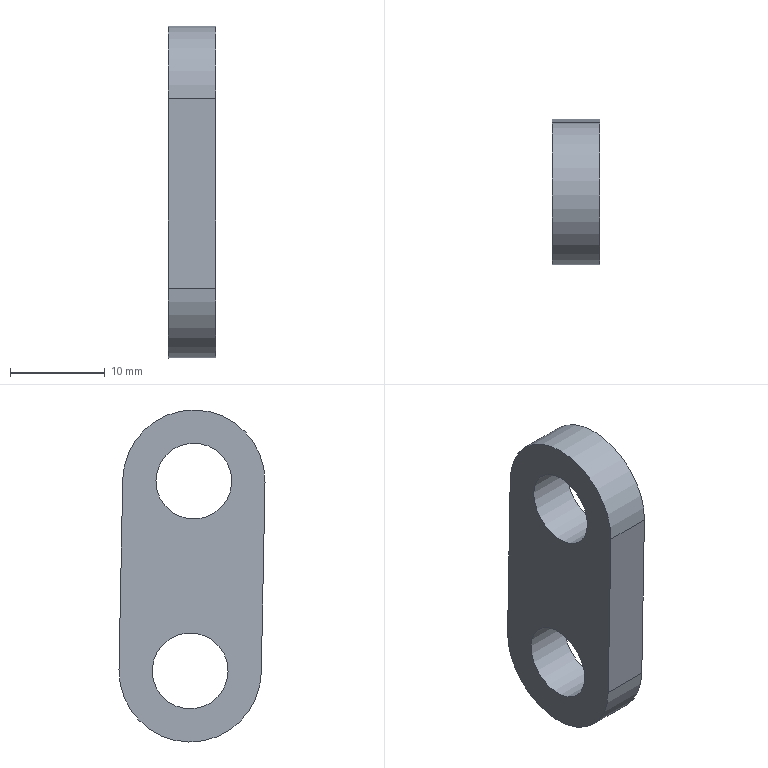Component | NX | LINK1_2 | 1 solid | 8 faces | box 5 x 15.39 x 35 mm | volume 1881 mm3 | plane 4 | cylinder 4 | commonest cylinder face diameters 15 x2 8 x2
STEP:
#1=CARTESIAN_POINT('',(0.,0.,0.));
#2=DIRECTION('',(0.,0.,1.));
#3=DIRECTION('',(1.,0.,0.));
#4=AXIS2_PLACEMENT_3D('',#1,#2,#3);
#5=CARTESIAN_POINT('',(4.61,-32.598,-197.455));
#6=VERTEX_POINT('',#5);
#7=CARTESIAN_POINT('',(4.61,-28.599,-197.377));
#8=DIRECTION('',(-1.,0.,0.));
#9=DIRECTION('',(0.,-0.9998,-0.01963));
#10=AXIS2_PLACEMENT_3D('',#7,#8,#9);
#11=CIRCLE('',#10,4.);
#12=CARTESIAN_POINT('',(4.61,-28.403,-207.375));
#13=DIRECTION('',(1.,0.,0.));
#14=DIRECTION('',(0.,0.9998,0.01963));
#15=AXIS2_PLACEMENT_3D('',#12,#13,#14);
#16=PLANE('',#15);
#17=CARTESIAN_POINT('',(-4.,10.));
#18=CARTESIAN_POINT('',(-4.,16.928));
#19=CARTESIAN_POINT('',(2.,13.464));
#20=CARTESIAN_POINT('',(8.,10.));
#21=CARTESIAN_POINT('',(2.,6.536));
#22=CARTESIAN_POINT('',(-4.,3.072));
#23=CARTESIAN_POINT('',(-4.,10.));
#24=(BOUNDED_CURVE()B_SPLINE_CURVE(2,(#17,#18,#19,#20,#21,#22,#23),.UNSPECIFIED.,.T.,.F.)B_SPLINE_CURVE_WITH_KNOTS((1,2,2,2,2,1),(-2.094,0.,2.094,4.189,6.283,8.378),.UNSPECIFIED.)CURVE()GEOMETRIC_REPRESENTATION_ITEM()RATIONAL_B_SPLINE_CURVE((1.,0.5,1.,0.5,1.,0.5,1.))REPRESENTATION_ITEM(''));
#25=(GEOMETRIC_REPRESENTATION_CONTEXT(2)PARAMETRIC_REPRESENTATION_CONTEXT()REPRESENTATION_CONTEXT('',''));
#26=DEFINITIONAL_REPRESENTATION('',(#24),#25);
#27=PCURVE('',#16,#26);
#28=CARTESIAN_POINT('',(4.61,-28.599,-197.377));
#29=DIRECTION('',(-1.,0.,0.));
#30=DIRECTION('',(0.,-0.9998,-0.01963));
#31=AXIS2_PLACEMENT_3D('',#28,#29,#30);
#32=CYLINDRICAL_SURFACE('',#31,4.);
#33=CARTESIAN_POINT('',(0.,0.));
#34=DIRECTION('',(1.,0.));
#35=VECTOR('',#34,1.);
#36=LINE('',#33,#35);
#37=(GEOMETRIC_REPRESENTATION_CONTEXT(2)PARAMETRIC_REPRESENTATION_CONTEXT()REPRESENTATION_CONTEXT('',''));
#38=DEFINITIONAL_REPRESENTATION('',(#36),#37);
#39=PCURVE('',#32,#38);
#40=SURFACE_CURVE('',#11,(#27,#39),.PCURVE_S1.);
#41=EDGE_CURVE('',#6,#6,#40,.T.);
#42=ORIENTED_EDGE('',*,*,#41,.T.);
#43=EDGE_LOOP('',(#42));
#44=FACE_BOUND('',#43,.T.);
#45=CARTESIAN_POINT('',(4.61,-32.206,-217.451));
#46=VERTEX_POINT('',#45);
#47=CARTESIAN_POINT('',(4.61,-28.206,-217.373));
#48=DIRECTION('',(-1.,0.,0.));
#49=DIRECTION('',(0.,-0.9998,-0.01963));
#50=AXIS2_PLACEMENT_3D('',#47,#48,#49);
#51=CIRCLE('',#50,4.);
#52=CARTESIAN_POINT('',(-4.,-10.));
#53=CARTESIAN_POINT('',(-4.,-3.072));
#54=CARTESIAN_POINT('',(2.,-6.536));
#55=CARTESIAN_POINT('',(8.,-10.));
#56=CARTESIAN_POINT('',(2.,-13.464));
#57=CARTESIAN_POINT('',(-4.,-16.928));
#58=CARTESIAN_POINT('',(-4.,-10.));
#59=(BOUNDED_CURVE()B_SPLINE_CURVE(2,(#52,#53,#54,#55,#56,#57,#58),.UNSPECIFIED.,.T.,.F.)B_SPLINE_CURVE_WITH_KNOTS((1,2,2,2,2,1),(-2.094,0.,2.094,4.189,6.283,8.378),.UNSPECIFIED.)CURVE()GEOMETRIC_REPRESENTATION_ITEM()RATIONAL_B_SPLINE_CURVE((1.,0.5,1.,0.5,1.,0.5,1.))REPRESENTATION_ITEM(''));
#60=(GEOMETRIC_REPRESENTATION_CONTEXT(2)PARAMETRIC_REPRESENTATION_CONTEXT()REPRESENTATION_CONTEXT('',''));
#61=DEFINITIONAL_REPRESENTATION('',(#59),#60);
#62=PCURVE('',#16,#61);
#63=CARTESIAN_POINT('',(4.61,-28.206,-217.373));
#64=DIRECTION('',(-1.,0.,0.));
#65=DIRECTION('',(0.,-0.9998,-0.01963));
#66=AXIS2_PLACEMENT_3D('',#63,#64,#65);
#67=CYLINDRICAL_SURFACE('',#66,4.);
#68=CARTESIAN_POINT('',(0.,0.));
#69=DIRECTION('',(1.,0.));
#70=VECTOR('',#69,1.);
#71=LINE('',#68,#70);
#72=(GEOMETRIC_REPRESENTATION_CONTEXT(2)PARAMETRIC_REPRESENTATION_CONTEXT()REPRESENTATION_CONTEXT('',''));
#73=DEFINITIONAL_REPRESENTATION('',(#71),#72);
#74=PCURVE('',#67,#73);
#75=SURFACE_CURVE('',#51,(#62,#74),.PCURVE_S1.);
#76=EDGE_CURVE('',#46,#46,#75,.T.);
#77=ORIENTED_EDGE('',*,*,#76,.T.);
#78=EDGE_LOOP('',(#77));
#79=FACE_BOUND('',#78,.T.);
#80=CARTESIAN_POINT('',(4.61,-21.1,-197.229));
#81=VERTEX_POINT('',#80);
#82=CARTESIAN_POINT('',(4.61,-36.098,-197.524));
#83=VERTEX_POINT('',#82);
#84=CARTESIAN_POINT('',(4.61,-28.599,-197.377));
#85=DIRECTION('',(1.,0.,0.));
#86=DIRECTION('',(0.,0.9998,0.01963));
#87=AXIS2_PLACEMENT_3D('',#84,#85,#86);
#88=CIRCLE('',#87,7.5);
#89=CARTESIAN_POINT('',(0.,10.));
#90=DIRECTION('',(1.,0.));
#91=AXIS2_PLACEMENT_2D('',#89,#90);
#92=CIRCLE('',#91,7.5);
#93=(GEOMETRIC_REPRESENTATION_CONTEXT(2)PARAMETRIC_REPRESENTATION_CONTEXT()REPRESENTATION_CONTEXT('',''));
#94=DEFINITIONAL_REPRESENTATION('',(#92),#93);
#95=PCURVE('',#16,#94);
#96=CARTESIAN_POINT('',(-0.3896,-28.599,-197.377));
#97=DIRECTION('',(1.,0.,0.));
#98=DIRECTION('',(0.,0.9998,0.01963));
#99=AXIS2_PLACEMENT_3D('',#96,#97,#98);
#100=CYLINDRICAL_SURFACE('',#99,7.5);
#101=CARTESIAN_POINT('',(0.,5.));
#102=DIRECTION('',(1.,0.));
#103=VECTOR('',#102,1.);
#104=LINE('',#101,#103);
#105=(GEOMETRIC_REPRESENTATION_CONTEXT(2)PARAMETRIC_REPRESENTATION_CONTEXT()REPRESENTATION_CONTEXT('',''));
#106=DEFINITIONAL_REPRESENTATION('',(#104),#105);
#107=PCURVE('',#100,#106);
#108=SURFACE_CURVE('',#88,(#95,#107),.PCURVE_S1.);
#109=EDGE_CURVE('',#81,#83,#108,.T.);
#110=ORIENTED_EDGE('',*,*,#109,.T.);
#111=CARTESIAN_POINT('',(4.61,-35.705,-217.52));
#112=VERTEX_POINT('',#111);
#113=CARTESIAN_POINT('',(4.61,-35.901,-207.522));
#114=DIRECTION('',(0.,-0.01963,0.9998));
#115=VECTOR('',#114,1.);
#116=LINE('',#113,#115);
#117=CARTESIAN_POINT('',(-7.5,-0.));
#118=DIRECTION('',(0.,1.));
#119=VECTOR('',#118,1.);
#120=LINE('',#117,#119);
#121=(GEOMETRIC_REPRESENTATION_CONTEXT(2)PARAMETRIC_REPRESENTATION_CONTEXT()REPRESENTATION_CONTEXT('',''));
#122=DEFINITIONAL_REPRESENTATION('',(#120),#121);
#123=PCURVE('',#16,#122);
#124=CARTESIAN_POINT('',(-0.3896,-35.901,-207.522));
#125=DIRECTION('',(0.,-0.9998,-0.01963));
#126=DIRECTION('',(1.,0.,0.));
#127=AXIS2_PLACEMENT_3D('',#124,#125,#126);
#128=PLANE('',#127);
#129=CARTESIAN_POINT('',(5.,0.));
#130=DIRECTION('',(0.,1.));
#131=VECTOR('',#130,1.);
#132=LINE('',#129,#131);
#133=(GEOMETRIC_REPRESENTATION_CONTEXT(2)PARAMETRIC_REPRESENTATION_CONTEXT()REPRESENTATION_CONTEXT('',''));
#134=DEFINITIONAL_REPRESENTATION('',(#132),#133);
#135=PCURVE('',#128,#134);
#136=SURFACE_CURVE('',#116,(#123,#135),.PCURVE_S1.);
#137=EDGE_CURVE('',#112,#83,#136,.T.);
#138=ORIENTED_EDGE('',*,*,#137,.F.);
#139=CARTESIAN_POINT('',(4.61,-20.708,-217.226));
#140=VERTEX_POINT('',#139);
#141=CARTESIAN_POINT('',(4.61,-28.206,-217.373));
#142=DIRECTION('',(1.,0.,0.));
#143=DIRECTION('',(0.,0.9998,0.01963));
#144=AXIS2_PLACEMENT_3D('',#141,#142,#143);
#145=CIRCLE('',#144,7.5);
#146=CARTESIAN_POINT('',(0.,-10.));
#147=DIRECTION('',(1.,0.));
#148=AXIS2_PLACEMENT_2D('',#146,#147);
#149=CIRCLE('',#148,7.5);
#150=(GEOMETRIC_REPRESENTATION_CONTEXT(2)PARAMETRIC_REPRESENTATION_CONTEXT()REPRESENTATION_CONTEXT('',''));
#151=DEFINITIONAL_REPRESENTATION('',(#149),#150);
#152=PCURVE('',#16,#151);
#153=CARTESIAN_POINT('',(-0.3896,-28.206,-217.373));
#154=DIRECTION('',(1.,0.,0.));
#155=DIRECTION('',(0.,0.9998,0.01963));
#156=AXIS2_PLACEMENT_3D('',#153,#154,#155);
#157=CYLINDRICAL_SURFACE('',#156,7.5);
#158=CARTESIAN_POINT('',(-0.,5.));
#159=DIRECTION('',(1.,0.));
#160=VECTOR('',#159,1.);
#161=LINE('',#158,#160);
#162=(GEOMETRIC_REPRESENTATION_CONTEXT(2)PARAMETRIC_REPRESENTATION_CONTEXT()REPRESENTATION_CONTEXT('',''));
#163=DEFINITIONAL_REPRESENTATION('',(#161),#162);
#164=PCURVE('',#157,#163);
#165=SURFACE_CURVE('',#145,(#152,#164),.PCURVE_S1.);
#166=EDGE_CURVE('',#112,#140,#165,.T.);
#167=ORIENTED_EDGE('',*,*,#166,.T.);
#168=CARTESIAN_POINT('',(4.61,-20.904,-207.228));
#169=DIRECTION('',(0.,0.01963,-0.9998));
#170=VECTOR('',#169,1.);
#171=LINE('',#168,#170);
#172=CARTESIAN_POINT('',(7.5,-0.));
#173=DIRECTION('',(0.,-1.));
#174=VECTOR('',#173,1.);
#175=LINE('',#172,#174);
#176=(GEOMETRIC_REPRESENTATION_CONTEXT(2)PARAMETRIC_REPRESENTATION_CONTEXT()REPRESENTATION_CONTEXT('',''));
#177=DEFINITIONAL_REPRESENTATION('',(#175),#176);
#178=PCURVE('',#16,#177);
#179=CARTESIAN_POINT('',(-0.3896,-20.904,-207.228));
#180=DIRECTION('',(0.,0.9998,0.01963));
#181=DIRECTION('',(-1.,0.,0.));
#182=AXIS2_PLACEMENT_3D('',#179,#180,#181);
#183=PLANE('',#182);
#184=CARTESIAN_POINT('',(-5.,0.));
#185=DIRECTION('',(0.,-1.));
#186=VECTOR('',#185,1.);
#187=LINE('',#184,#186);
#188=(GEOMETRIC_REPRESENTATION_CONTEXT(2)PARAMETRIC_REPRESENTATION_CONTEXT()REPRESENTATION_CONTEXT('',''));
#189=DEFINITIONAL_REPRESENTATION('',(#187),#188);
#190=PCURVE('',#183,#189);
#191=SURFACE_CURVE('',#171,(#178,#190),.PCURVE_S1.);
#192=EDGE_CURVE('',#81,#140,#191,.T.);
#193=ORIENTED_EDGE('',*,*,#192,.F.);
#194=EDGE_LOOP('',(#110,#138,#167,#193));
#195=FACE_BOUND('',#194,.T.);
#196=ADVANCED_FACE('',(#44,#79,#195),#16,.T.);
#197=ORIENTED_EDGE('',*,*,#137,.T.);
#198=CARTESIAN_POINT('',(-0.3896,-36.098,-197.524));
#199=VERTEX_POINT('',#198);
#200=CARTESIAN_POINT('',(-0.3896,-36.098,-197.524));
#201=DIRECTION('',(-1.,0.,0.));
#202=VECTOR('',#201,1.);
#203=LINE('',#200,#202);
#204=CARTESIAN_POINT('',(0.,10.));
#205=DIRECTION('',(-1.,0.));
#206=VECTOR('',#205,1.);
#207=LINE('',#204,#206);
#208=(GEOMETRIC_REPRESENTATION_CONTEXT(2)PARAMETRIC_REPRESENTATION_CONTEXT()REPRESENTATION_CONTEXT('',''));
#209=DEFINITIONAL_REPRESENTATION('',(#207),#208);
#210=PCURVE('',#128,#209);
#211=CARTESIAN_POINT('',(3.142,0.));
#212=DIRECTION('',(0.,-1.));
#213=VECTOR('',#212,1.);
#214=LINE('',#211,#213);
#215=(GEOMETRIC_REPRESENTATION_CONTEXT(2)PARAMETRIC_REPRESENTATION_CONTEXT()REPRESENTATION_CONTEXT('',''));
#216=DEFINITIONAL_REPRESENTATION('',(#214),#215);
#217=PCURVE('',#100,#216);
#218=SURFACE_CURVE('',#203,(#210,#217),.PCURVE_S1.);
#219=EDGE_CURVE('',#83,#199,#218,.T.);
#220=ORIENTED_EDGE('',*,*,#219,.T.);
#221=CARTESIAN_POINT('',(-0.3896,-35.705,-217.52));
#222=VERTEX_POINT('',#221);
#223=CARTESIAN_POINT('',(-0.3896,-35.901,-207.522));
#224=DIRECTION('',(0.,0.01963,-0.9998));
#225=VECTOR('',#224,1.);
#226=LINE('',#223,#225);
#227=CARTESIAN_POINT('',(0.,0.));
#228=DIRECTION('',(0.,-1.));
#229=VECTOR('',#228,1.);
#230=LINE('',#227,#229);
#231=(GEOMETRIC_REPRESENTATION_CONTEXT(2)PARAMETRIC_REPRESENTATION_CONTEXT()REPRESENTATION_CONTEXT('',''));
#232=DEFINITIONAL_REPRESENTATION('',(#230),#231);
#233=PCURVE('',#128,#232);
#234=CARTESIAN_POINT('',(-0.3896,-28.403,-207.375));
#235=DIRECTION('',(-1.,0.,0.));
#236=DIRECTION('',(0.,-0.9998,-0.01963));
#237=AXIS2_PLACEMENT_3D('',#234,#235,#236);
#238=PLANE('',#237);
#239=CARTESIAN_POINT('',(7.5,-0.));
#240=DIRECTION('',(0.,-1.));
#241=VECTOR('',#240,1.);
#242=LINE('',#239,#241);
#243=(GEOMETRIC_REPRESENTATION_CONTEXT(2)PARAMETRIC_REPRESENTATION_CONTEXT()REPRESENTATION_CONTEXT('',''));
#244=DEFINITIONAL_REPRESENTATION('',(#242),#243);
#245=PCURVE('',#238,#244);
#246=SURFACE_CURVE('',#226,(#233,#245),.PCURVE_S1.);
#247=EDGE_CURVE('',#199,#222,#246,.T.);
#248=ORIENTED_EDGE('',*,*,#247,.T.);
#249=CARTESIAN_POINT('',(-0.3896,-35.705,-217.52));
#250=DIRECTION('',(1.,0.,0.));
#251=VECTOR('',#250,1.);
#252=LINE('',#249,#251);
#253=CARTESIAN_POINT('',(0.,-10.));
#254=DIRECTION('',(1.,0.));
#255=VECTOR('',#254,1.);
#256=LINE('',#253,#255);
#257=(GEOMETRIC_REPRESENTATION_CONTEXT(2)PARAMETRIC_REPRESENTATION_CONTEXT()REPRESENTATION_CONTEXT('',''));
#258=DEFINITIONAL_REPRESENTATION('',(#256),#257);
#259=PCURVE('',#128,#258);
#260=CARTESIAN_POINT('',(3.142,0.));
#261=DIRECTION('',(0.,1.));
#262=VECTOR('',#261,1.);
#263=LINE('',#260,#262);
#264=(GEOMETRIC_REPRESENTATION_CONTEXT(2)PARAMETRIC_REPRESENTATION_CONTEXT()REPRESENTATION_CONTEXT('',''));
#265=DEFINITIONAL_REPRESENTATION('',(#263),#264);
#266=PCURVE('',#157,#265);
#267=SURFACE_CURVE('',#252,(#259,#266),.PCURVE_S1.);
#268=EDGE_CURVE('',#222,#112,#267,.T.);
#269=ORIENTED_EDGE('',*,*,#268,.T.);
#270=EDGE_LOOP('',(#197,#220,#248,#269));
#271=FACE_BOUND('',#270,.T.);
#272=ADVANCED_FACE('',(#271),#128,.T.);
#273=CARTESIAN_POINT('',(-0.3896,-32.598,-197.455));
#274=VERTEX_POINT('',#273);
#275=CARTESIAN_POINT('',(-0.3896,-28.599,-197.377));
#276=DIRECTION('',(-1.,0.,0.));
#277=DIRECTION('',(0.,-0.9998,-0.01963));
#278=AXIS2_PLACEMENT_3D('',#275,#276,#277);
#279=CIRCLE('',#278,4.);
#280=CARTESIAN_POINT('',(-0.,10.));
#281=DIRECTION('',(1.,0.));
#282=AXIS2_PLACEMENT_2D('',#280,#281);
#283=CIRCLE('',#282,4.);
#284=(GEOMETRIC_REPRESENTATION_CONTEXT(2)PARAMETRIC_REPRESENTATION_CONTEXT()REPRESENTATION_CONTEXT('',''));
#285=DEFINITIONAL_REPRESENTATION('',(#283),#284);
#286=PCURVE('',#238,#285);
#287=CARTESIAN_POINT('',(0.,5.));
#288=DIRECTION('',(1.,0.));
#289=VECTOR('',#288,1.);
#290=LINE('',#287,#289);
#291=(GEOMETRIC_REPRESENTATION_CONTEXT(2)PARAMETRIC_REPRESENTATION_CONTEXT()REPRESENTATION_CONTEXT('',''));
#292=DEFINITIONAL_REPRESENTATION('',(#290),#291);
#293=PCURVE('',#32,#292);
#294=SURFACE_CURVE('',#279,(#286,#293),.PCURVE_S1.);
#295=EDGE_CURVE('',#274,#274,#294,.T.);
#296=ORIENTED_EDGE('',*,*,#295,.F.);
#297=EDGE_LOOP('',(#296));
#298=FACE_BOUND('',#297,.T.);
#299=CARTESIAN_POINT('',(-0.3896,-32.206,-217.451));
#300=VERTEX_POINT('',#299);
#301=CARTESIAN_POINT('',(-0.3896,-28.206,-217.373));
#302=DIRECTION('',(-1.,0.,0.));
#303=DIRECTION('',(0.,-0.9998,-0.01963));
#304=AXIS2_PLACEMENT_3D('',#301,#302,#303);
#305=CIRCLE('',#304,4.);
#306=CARTESIAN_POINT('',(-0.,-10.));
#307=DIRECTION('',(1.,0.));
#308=AXIS2_PLACEMENT_2D('',#306,#307);
#309=CIRCLE('',#308,4.);
#310=(GEOMETRIC_REPRESENTATION_CONTEXT(2)PARAMETRIC_REPRESENTATION_CONTEXT()REPRESENTATION_CONTEXT('',''));
#311=DEFINITIONAL_REPRESENTATION('',(#309),#310);
#312=PCURVE('',#238,#311);
#313=CARTESIAN_POINT('',(0.,5.));
#314=DIRECTION('',(1.,0.));
#315=VECTOR('',#314,1.);
#316=LINE('',#313,#315);
#317=(GEOMETRIC_REPRESENTATION_CONTEXT(2)PARAMETRIC_REPRESENTATION_CONTEXT()REPRESENTATION_CONTEXT('',''));
#318=DEFINITIONAL_REPRESENTATION('',(#316),#317);
#319=PCURVE('',#67,#318);
#320=SURFACE_CURVE('',#305,(#312,#319),.PCURVE_S1.);
#321=EDGE_CURVE('',#300,#300,#320,.T.);
#322=ORIENTED_EDGE('',*,*,#321,.F.);
#323=EDGE_LOOP('',(#322));
#324=FACE_BOUND('',#323,.T.);
#325=ORIENTED_EDGE('',*,*,#247,.F.);
#326=CARTESIAN_POINT('',(-0.3896,-21.1,-197.229));
#327=VERTEX_POINT('',#326);
#328=CARTESIAN_POINT('',(-0.3896,-28.599,-197.377));
#329=DIRECTION('',(-1.,0.,0.));
#330=DIRECTION('',(0.,-0.9998,-0.01963));
#331=AXIS2_PLACEMENT_3D('',#328,#329,#330);
#332=CIRCLE('',#331,7.5);
#333=CARTESIAN_POINT('',(-0.,10.));
#334=DIRECTION('',(1.,-0.));
#335=AXIS2_PLACEMENT_2D('',#333,#334);
#336=CIRCLE('',#335,7.5);
#337=(GEOMETRIC_REPRESENTATION_CONTEXT(2)PARAMETRIC_REPRESENTATION_CONTEXT()REPRESENTATION_CONTEXT('',''));
#338=DEFINITIONAL_REPRESENTATION('',(#336),#337);
#339=PCURVE('',#238,#338);
#340=CARTESIAN_POINT('',(3.142,0.));
#341=DIRECTION('',(-1.,0.));
#342=VECTOR('',#341,1.);
#343=LINE('',#340,#342);
#344=(GEOMETRIC_REPRESENTATION_CONTEXT(2)PARAMETRIC_REPRESENTATION_CONTEXT()REPRESENTATION_CONTEXT('',''));
#345=DEFINITIONAL_REPRESENTATION('',(#343),#344);
#346=PCURVE('',#100,#345);
#347=SURFACE_CURVE('',#332,(#339,#346),.PCURVE_S1.);
#348=EDGE_CURVE('',#199,#327,#347,.T.);
#349=ORIENTED_EDGE('',*,*,#348,.T.);
#350=CARTESIAN_POINT('',(-0.3896,-20.708,-217.226));
#351=VERTEX_POINT('',#350);
#352=CARTESIAN_POINT('',(-0.3896,-20.904,-207.228));
#353=DIRECTION('',(0.,-0.01963,0.9998));
#354=VECTOR('',#353,1.);
#355=LINE('',#352,#354);
#356=CARTESIAN_POINT('',(-7.5,-0.));
#357=DIRECTION('',(0.,1.));
#358=VECTOR('',#357,1.);
#359=LINE('',#356,#358);
#360=(GEOMETRIC_REPRESENTATION_CONTEXT(2)PARAMETRIC_REPRESENTATION_CONTEXT()REPRESENTATION_CONTEXT('',''));
#361=DEFINITIONAL_REPRESENTATION('',(#359),#360);
#362=PCURVE('',#238,#361);
#363=CARTESIAN_POINT('',(0.,0.));
#364=DIRECTION('',(0.,1.));
#365=VECTOR('',#364,1.);
#366=LINE('',#363,#365);
#367=(GEOMETRIC_REPRESENTATION_CONTEXT(2)PARAMETRIC_REPRESENTATION_CONTEXT()REPRESENTATION_CONTEXT('',''));
#368=DEFINITIONAL_REPRESENTATION('',(#366),#367);
#369=PCURVE('',#183,#368);
#370=SURFACE_CURVE('',#355,(#362,#369),.PCURVE_S1.);
#371=EDGE_CURVE('',#351,#327,#370,.T.);
#372=ORIENTED_EDGE('',*,*,#371,.F.);
#373=CARTESIAN_POINT('',(-0.3896,-28.206,-217.373));
#374=DIRECTION('',(-1.,0.,0.));
#375=DIRECTION('',(0.,-0.9998,-0.01963));
#376=AXIS2_PLACEMENT_3D('',#373,#374,#375);
#377=CIRCLE('',#376,7.5);
#378=CARTESIAN_POINT('',(-0.,-10.));
#379=DIRECTION('',(1.,-0.));
#380=AXIS2_PLACEMENT_2D('',#378,#379);
#381=CIRCLE('',#380,7.5);
#382=(GEOMETRIC_REPRESENTATION_CONTEXT(2)PARAMETRIC_REPRESENTATION_CONTEXT()REPRESENTATION_CONTEXT('',''));
#383=DEFINITIONAL_REPRESENTATION('',(#381),#382);
#384=PCURVE('',#238,#383);
#385=CARTESIAN_POINT('',(9.425,0.));
#386=DIRECTION('',(-1.,0.));
#387=VECTOR('',#386,1.);
#388=LINE('',#385,#387);
#389=(GEOMETRIC_REPRESENTATION_CONTEXT(2)PARAMETRIC_REPRESENTATION_CONTEXT()REPRESENTATION_CONTEXT('',''));
#390=DEFINITIONAL_REPRESENTATION('',(#388),#389);
#391=PCURVE('',#157,#390);
#392=SURFACE_CURVE('',#377,(#384,#391),.PCURVE_S1.);
#393=EDGE_CURVE('',#351,#222,#392,.T.);
#394=ORIENTED_EDGE('',*,*,#393,.T.);
#395=EDGE_LOOP('',(#325,#349,#372,#394));
#396=FACE_BOUND('',#395,.T.);
#397=ADVANCED_FACE('',(#298,#324,#396),#238,.T.);
#398=ORIENTED_EDGE('',*,*,#371,.T.);
#399=CARTESIAN_POINT('',(-0.3896,-21.1,-197.229));
#400=DIRECTION('',(1.,0.,0.));
#401=VECTOR('',#400,1.);
#402=LINE('',#399,#401);
#403=CARTESIAN_POINT('',(0.,10.));
#404=DIRECTION('',(-1.,0.));
#405=VECTOR('',#404,1.);
#406=LINE('',#403,#405);
#407=(GEOMETRIC_REPRESENTATION_CONTEXT(2)PARAMETRIC_REPRESENTATION_CONTEXT()REPRESENTATION_CONTEXT('',''));
#408=DEFINITIONAL_REPRESENTATION('',(#406),#407);
#409=PCURVE('',#183,#408);
#410=CARTESIAN_POINT('',(0.,0.));
#411=DIRECTION('',(0.,1.));
#412=VECTOR('',#411,1.);
#413=LINE('',#410,#412);
#414=(GEOMETRIC_REPRESENTATION_CONTEXT(2)PARAMETRIC_REPRESENTATION_CONTEXT()REPRESENTATION_CONTEXT('',''));
#415=DEFINITIONAL_REPRESENTATION('',(#413),#414);
#416=PCURVE('',#100,#415);
#417=SURFACE_CURVE('',#402,(#409,#416),.PCURVE_S1.);
#418=EDGE_CURVE('',#327,#81,#417,.T.);
#419=ORIENTED_EDGE('',*,*,#418,.T.);
#420=ORIENTED_EDGE('',*,*,#192,.T.);
#421=CARTESIAN_POINT('',(-0.3896,-20.708,-217.226));
#422=DIRECTION('',(-1.,0.,0.));
#423=VECTOR('',#422,1.);
#424=LINE('',#421,#423);
#425=CARTESIAN_POINT('',(0.,-10.));
#426=DIRECTION('',(1.,0.));
#427=VECTOR('',#426,1.);
#428=LINE('',#425,#427);
#429=(GEOMETRIC_REPRESENTATION_CONTEXT(2)PARAMETRIC_REPRESENTATION_CONTEXT()REPRESENTATION_CONTEXT('',''));
#430=DEFINITIONAL_REPRESENTATION('',(#428),#429);
#431=PCURVE('',#183,#430);
#432=CARTESIAN_POINT('',(6.283,0.));
#433=DIRECTION('',(0.,-1.));
#434=VECTOR('',#433,1.);
#435=LINE('',#432,#434);
#436=(GEOMETRIC_REPRESENTATION_CONTEXT(2)PARAMETRIC_REPRESENTATION_CONTEXT()REPRESENTATION_CONTEXT('',''));
#437=DEFINITIONAL_REPRESENTATION('',(#435),#436);
#438=PCURVE('',#157,#437);
#439=SURFACE_CURVE('',#424,(#431,#438),.PCURVE_S1.);
#440=EDGE_CURVE('',#140,#351,#439,.T.);
#441=ORIENTED_EDGE('',*,*,#440,.T.);
#442=EDGE_LOOP('',(#398,#419,#420,#441));
#443=FACE_BOUND('',#442,.T.);
#444=ADVANCED_FACE('',(#443),#183,.T.);
#445=ORIENTED_EDGE('',*,*,#418,.F.);
#446=ORIENTED_EDGE('',*,*,#348,.F.);
#447=ORIENTED_EDGE('',*,*,#219,.F.);
#448=ORIENTED_EDGE('',*,*,#109,.F.);
#449=EDGE_LOOP('',(#445,#446,#447,#448));
#450=FACE_BOUND('',#449,.T.);
#451=ADVANCED_FACE('',(#450),#100,.T.);
#452=ORIENTED_EDGE('',*,*,#166,.F.);
#453=ORIENTED_EDGE('',*,*,#268,.F.);
#454=ORIENTED_EDGE('',*,*,#393,.F.);
#455=ORIENTED_EDGE('',*,*,#440,.F.);
#456=EDGE_LOOP('',(#452,#453,#454,#455));
#457=FACE_BOUND('',#456,.T.);
#458=ADVANCED_FACE('',(#457),#157,.T.);
#459=ORIENTED_EDGE('',*,*,#321,.F.);
#460=CARTESIAN_POINT('',(4.61,-32.206,-217.451));
#461=CARTESIAN_POINT('',(-0.3896,-32.206,-217.451));
#462=B_SPLINE_CURVE_WITH_KNOTS('',1,(#460,#461),.UNSPECIFIED.,.F.,.F.,(2,2),(0.,5.),.PIECEWISE_BEZIER_KNOTS.);
#463=CARTESIAN_POINT('',(0.,0.));
#464=DIRECTION('',(0.,1.));
#465=VECTOR('',#464,1.);
#466=LINE('',#463,#465);
#467=(GEOMETRIC_REPRESENTATION_CONTEXT(2)PARAMETRIC_REPRESENTATION_CONTEXT()REPRESENTATION_CONTEXT('',''));
#468=DEFINITIONAL_REPRESENTATION('',(#466),#467);
#469=PCURVE('',#67,#468);
#470=CARTESIAN_POINT('',(6.283,0.));
#471=DIRECTION('',(0.,1.));
#472=VECTOR('',#471,1.);
#473=LINE('',#470,#472);
#474=(GEOMETRIC_REPRESENTATION_CONTEXT(2)PARAMETRIC_REPRESENTATION_CONTEXT()REPRESENTATION_CONTEXT('',''));
#475=DEFINITIONAL_REPRESENTATION('',(#473),#474);
#476=PCURVE('',#67,#475);
#477=SEAM_CURVE('',#462,(#469,#476),.PCURVE_S1.);
#478=EDGE_CURVE('',#46,#300,#477,.T.);
#479=ORIENTED_EDGE('',*,*,#478,.F.);
#480=ORIENTED_EDGE('',*,*,#76,.T.);
#481=ORIENTED_EDGE('',*,*,#478,.T.);
#482=EDGE_LOOP('',(#459,#479,#480,#481));
#483=FACE_BOUND('',#482,.F.);
#484=ADVANCED_FACE('',(#483),#67,.F.);
#485=ORIENTED_EDGE('',*,*,#295,.F.);
#486=CARTESIAN_POINT('',(4.61,-32.598,-197.455));
#487=CARTESIAN_POINT('',(-0.3896,-32.598,-197.455));
#488=B_SPLINE_CURVE_WITH_KNOTS('',1,(#486,#487),.UNSPECIFIED.,.F.,.F.,(2,2),(0.,5.),.PIECEWISE_BEZIER_KNOTS.);
#489=CARTESIAN_POINT('',(0.,0.));
#490=DIRECTION('',(0.,1.));
#491=VECTOR('',#490,1.);
#492=LINE('',#489,#491);
#493=(GEOMETRIC_REPRESENTATION_CONTEXT(2)PARAMETRIC_REPRESENTATION_CONTEXT()REPRESENTATION_CONTEXT('',''));
#494=DEFINITIONAL_REPRESENTATION('',(#492),#493);
#495=PCURVE('',#32,#494);
#496=CARTESIAN_POINT('',(6.283,0.));
#497=DIRECTION('',(0.,1.));
#498=VECTOR('',#497,1.);
#499=LINE('',#496,#498);
#500=(GEOMETRIC_REPRESENTATION_CONTEXT(2)PARAMETRIC_REPRESENTATION_CONTEXT()REPRESENTATION_CONTEXT('',''));
#501=DEFINITIONAL_REPRESENTATION('',(#499),#500);
#502=PCURVE('',#32,#501);
#503=SEAM_CURVE('',#488,(#495,#502),.PCURVE_S1.);
#504=EDGE_CURVE('',#6,#274,#503,.T.);
#505=ORIENTED_EDGE('',*,*,#504,.F.);
#506=ORIENTED_EDGE('',*,*,#41,.T.);
#507=ORIENTED_EDGE('',*,*,#504,.T.);
#508=EDGE_LOOP('',(#485,#505,#506,#507));
#509=FACE_BOUND('',#508,.F.);
#510=ADVANCED_FACE('',(#509),#32,.F.);
#511=CLOSED_SHELL('',(#196,#272,#397,#444,#451,#458,#484,#510));
#512=MANIFOLD_SOLID_BREP('',#511);
#513=(LENGTH_UNIT()NAMED_UNIT(*)SI_UNIT(.MILLI.,.METRE.));
#514=UNCERTAINTY_MEASURE_WITH_UNIT(LENGTH_MEASURE(0.000002),#513,'','');
#515=(NAMED_UNIT(*)PLANE_ANGLE_UNIT()SI_UNIT($,.RADIAN.));
#516=(NAMED_UNIT(*)SI_UNIT($,.STERADIAN.)SOLID_ANGLE_UNIT());
#517=(GEOMETRIC_REPRESENTATION_CONTEXT(3)GLOBAL_UNCERTAINTY_ASSIGNED_CONTEXT((#514))GLOBAL_UNIT_ASSIGNED_CONTEXT((#513,#515,#516))REPRESENTATION_CONTEXT('',''));
#518=ADVANCED_BREP_SHAPE_REPRESENTATION('',(#4,#512),#517);